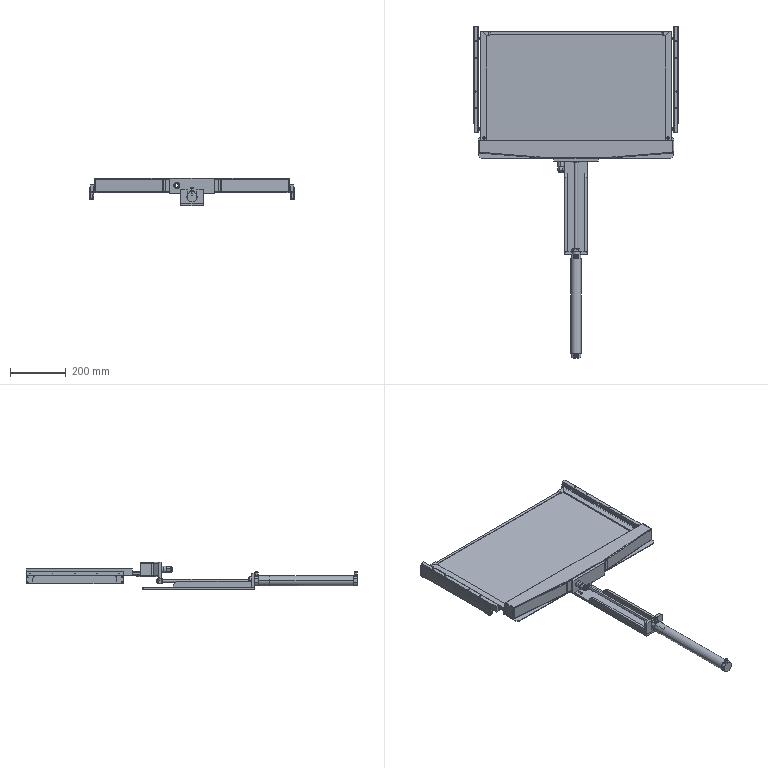Assembly | SolidWorks | mm | 22 component files | 33 solids | 974 faces | box 734 x 1190 x 97 mm | volume 3303453 mm3 | plane 403 | cylinder 333 | cone 192 | torus 22 | spline 16 | sphere 8 | commonest cylinder face diameters 4.5 x44 10 x34 2.5 x28 8 x26 4 x26 3.3 x22 3.4 x20 2.459 x16
Bill of materials:
A4-BPF02-3-PP-L | 4 |  | Short, large-diameter cylinder with chamfered ends. One end face has concentric stepped rings or a recess. A smaller coaxial round shaft sticks out of that face and carries a hex-shaped feature partway along it.
A4-MLCNLSS12-3-L | 1 |  | Hollow round part with a through bore. A hexagonal flats section sits in the middle. A slightly tapered cylindrical spigot with a chamfered end runs from one side. The other side has a short cylindrical neck with a step or groove and a flange-like ring.
A4-MLCNLSS4-1-L | 2 |  | Axially symmetric part with a through bore. From top to bottom: a short cylindrical collar, a narrow groove, a slightly larger ring/flange, a hexagonal body, then a cylindrical shank that tapers slightly and has a chamfer at the lower end.
A4-NA2-N16-L | 1 |  | Long, flat rectangular bar with rounded corners and edges. It has two small through holes near each end.
A4-SDA 32X300-KC-L1 | 1 |  | Long cylindrical rod. Near each end there are flats or notches with small cross holes. One end has a stepped, reduced-diameter tip with a polygonal (hex-like) section.
A4-SDA 32X300-KC-L2 | 1 |  | Long, slender round rod with a short, larger-diameter cylindrical head at one end. The other end has two small collar or hex-like features with a short tip.
AUTO-SpinDryWashing-01-03000001 | 1 | AISI 316 Stainless Steel Sheet (SS) | Elongated flat base plate. One end has an upright block with a U-shaped notch. Two raised rails run along the long edges for part of the length. The thinner opposite end has four slotted holes.
AUTO-SpinDryWashing-01-03000002 | 1 | AISI 316 Stainless Steel Sheet (SS) | Long rectangular box-section beam with rounded edges sitting on a wider flat base flange with chamfered ends. A plate wraps around the middle and carries a projecting cylindrical boss and a tab with a slot below it.
AUTO-SpinDryWashing-01-03000003 | 1 | Glass | Thin, flat rectangular plate with no visible holes or features.
AUTO-SpinDryWashing-01-03000004 | 1 | AISI 316 Stainless Steel Sheet (SS) | Long bar with a stepped, notched cross-section. A row of small holes runs along the top face. Both ends have rebated steps with small holes.
AUTO-SpinDryWashing-01-03000005 | 1 | AISI 304 | Long bar with a channel-like cross-section that has a rectangular groove along one side. Two larger holes sit near one end and small holes near the other. The corners at the ends are chamfered.
AUTO-SpinDryWashing-01-03000006 | 1 | AISI 304 | Long, slender bar with a side-notched cross-section and a round hole visible through the end face. The ends are stepped tabs with small holes and chamfered corners.
AUTO-SpinDryWashing-01-03000007 | 1 | AISI 304 | Long bar with a rectangular groove along one side. Two holes sit near one end. The ends have chamfered corners.
AUTO-SpinDryWashing-01-03000008 | 1 | AISI 304 | Long straight prismatic bar. Its constant cross-section is mostly rectangular, and one long side has a stepped profile: a narrow upper rib, a recessed longitudinal channel, and a lower lip. The top face has a row of small holes.
AUTO-SpinDryWashing-01-03000009 | 2 | AISI 304 | Thin, flat, elongated plate shaped like a shallow U or bridge. A long rectangular cutout along one long edge, with rounded inner corners, leaves a narrow top strip joining two wider end pads. The plate has small holes in the end pads and along the strip.
'- | 1 | AISI 304 | Long straight bar of constant cross-section. The profile is a rectangle with a stepped edge along one side: two projecting lips with a shallow recess between them, running the full length. Holes are spaced along the top face and along one side face.
Mates:
1. coincident | AUTO-SpinDryWashing-01-03000001-1 face at (40, 0, 58) dir (0, -1, 0) | A4-SDA 32X300-KC-L-1/A4-SDA 32X300-KC-L1-1 face at (0, 0, 31) dir (0, 1, 0)
2. concentric | AUTO-SpinDryWashing-01-03000001-1 face at (0, 60, 31) dir (0, -1, 0) r 14.5 | A4-SDA 32X300-KC-L-1/A4-SDA 32X300-KC-L1-1 face at (0, 20, 31) dir (0, -1, 0) r 13.5
3. parallel | AUTO-SpinDryWashing-01-03000001-1 face at (0, 0, 58) dir (0, 0, 1) | A4-SDA 32X300-KC-L-1/A4-SDA 32X300-KC-L1-1 face at (10, 0, 50) dir (0, 0, 1)
4. coincident | AUTO-SpinDryWashing-01-03000002-1 plane at (0, 343, 72) dir (-1, 0, 0) | assembly plane at (0, 0, 0) dir (1, 0, 0)
5. parallel | AUTO-SpinDryWashing-01-03000001-1 face at (40, 0, 58) dir (0, -1, 0) | AUTO-SpinDryWashing-01-03000002-1 face at (0, 333, 72) dir (0, -1, 0)
6. coincident | A4-SDA 32X300-KC-L-1/A4-SDA 32X300-KC-L2-1 face at (0, 343, 31) dir (0, -1, 0) | AUTO-SpinDryWashing-01-03000002-1 face at (0, 343, 72) dir (0, 1, 0)
7. coincident | AUTO-SpinDryWashing-01-03000002-1 face at (0, 343, 47) dir (0, 0, 1) | AUTO-SpinDryWashing-01-03000004-1 face at (-335, 423, 47) dir (0, 0, -1)
8. coincident | AUTO-SpinDryWashing-01-03000002-1 face at (350, 423, 45) dir (0, 1, 0) | AUTO-SpinDryWashing-01-03000004-1 face at (335, 423, 63) dir (0, 1, 0)
9. coincident | AUTO-SpinDryWashing-01-03000004-1 plane at (0, 408, 53) dir (1, 0, 0) | assembly plane at (0, 0, 0) dir (1, 0, 0)
10. coincident | AUTO-SpinDryWashing-01-03000004-1 face at (-335, 388, 60) dir (0, 1, 0) | AUTO-SpinDryWashing-01-03000003-1 face at (-325, 388, 60) dir (0, -1, 0)
11. coincident | AUTO-SpinDryWashing-01-03000004-1 face at (-335, 423, 55) dir (0, 0, 1) | AUTO-SpinDryWashing-01-03000003-1 face at (0, 588, 55) dir (0, 0, -1)
12. coincident | AUTO-SpinDryWashing-01-03000003-1 plane at (0, 588, 55) dir (1, 0, 0) | assembly plane at (0, 0, 0) dir (1, 0, 0)
13. coincident | AUTO-SpinDryWashing-01-03000003-1 face at (325, 788, 60) dir (1, 0, 0) | AUTO-SpinDryWashing-01-03000005-1 face at (325, 798, 63) dir (-1, 0, 0)
14. coincident | AUTO-SpinDryWashing-01-03000003-1 face at (0, 588, 60) dir (0, 0, 1) | AUTO-SpinDryWashing-01-03000005-1 face at (335, 798, 60) dir (0, 0, -1)
15. coincident | AUTO-SpinDryWashing-01-03000003-1 face at (-325, 788, 60) dir (0, 1, 0) | AUTO-SpinDryWashing-01-03000006-1 face at (335, 788, 50) dir (0, -1, 0)
16. coincident | AUTO-SpinDryWashing-01-03000003-1 face at (0, 588, 55) dir (0, 0, -1) | AUTO-SpinDryWashing-01-03000006-1 face at (335, 798, 55) dir (0, 0, 1)
17. coincident | AUTO-SpinDryWashing-01-03000005-1 face at (335, 798, 52) dir (-0.7071, 0.7071, 0) | AUTO-SpinDryWashing-01-03000006-1 face at (335, 798, 50) dir (0.7071, -0.7071, 0)
18. coincident | AUTO-SpinDryWashing-01-03000003-1 face at (-325, 788, 60) dir (-1, 0, 0) | AUTO-SpinDryWashing-01-03000007-1 face at (-325, 378, 63) dir (1, 0, 0)
19. coincident | AUTO-SpinDryWashing-01-03000003-1 face at (0, 588, 55) dir (0, 0, -1) | AUTO-SpinDryWashing-01-03000007-1 face at (-335, 378, 55) dir (0, 0, 1)
20. coincident | AUTO-SpinDryWashing-01-03000006-1 face at (-335, 798, 50) dir (-0.7071, -0.7071, 0) | AUTO-SpinDryWashing-01-03000007-1 face at (-335, 798, 52) dir (0.7071, 0.7071, 0)
21. distance | AUTO-SpinDryWashing-01-03000001-1 face at (-40, 400, 8) dir (0, 1, 0) | AUTO-SpinDryWashing-01-03000008-3 face at (-357, 818, 57.5) dir (0, 1, 0)
22. coincident | AUTO-SpinDryWashing-01-03000009-1 face at (365, 643, 42.5) dir (-1, 0, 0) | A4-NA2-N16-L-1 face at (365, 748, 35) dir (1, 0, 0)
23. coincident | AUTO-SpinDryWashing-01-03000009-1 face at (367, 468, 42.5) dir (0, -1, 0) | A4-NA2-N16-L-1 face at (365, 468, 20) dir (0, -1, 0)
24. coincident | A4-NA2-N16-L-1 face at (365, 818, 20) dir (0, 0, -1) | A4-NA2-N16-L-2 face at (-365, 468, 20) dir (0, 0, -1)
25. coincident | A4-NA2-N16-L-1 face at (365, 818, 50) dir (0, 1, 0) | A4-NA2-N16-L-2 face at (-365, 818, 20) dir (0, 1, 0)
26. distance | AUTO-SpinDryWashing-01-03000008-3 face at (-349, 468, 57.5) dir (1, 0, 0) | AUTO-SpinDryWashing-01-03000007-1 edge at (-335, 798, 65) dir (0, 0, -1)
27. coincident | AUTO-SpinDryWashing-01-03000008-3 face at (-365, 468, 57.5) dir (-1, 0, 0) | AUTO-SpinDryWashing-01-03000009-2 face at (-365, 643, 42.5) dir (1, 0, 0)
28. coincident | AUTO-SpinDryWashing-01-03000008-3 face at (-357, 818, 57.5) dir (0, 1, 0) | AUTO-SpinDryWashing-01-03000009-2 face at (-365, 818, 42.5) dir (0, 1, 0)
29. coincident | AUTO-SpinDryWashing-01-03000008-3 face at (-357, 468, 65) dir (0, 0, 1) | AUTO-SpinDryWashing-01-03000009-2 face at (-365, 643, 65) dir (0, 0, 1)
30. coincident | AUTO-SpinDryWashing-01-03000009-2 face at (-365, 643, 42.5) dir (1, 0, 0) | A4-NA2-N16-L-2 face at (-365, 748, 35) dir (-1, 0, 0)
31. coincident | AUTO-SpinDryWashing-01-03000008-3 face at (-357, 818, 57.5) dir (0, 1, 0) | A4-NA2-N16-L-2 face at (-365, 818, 20) dir (0, 1, 0)
32. coincident | AUTO-SpinDryWashing-01-03000009-2 face at (-365, 643, 20) dir (0, 0, -1) | A4-NA2-N16-L-2 face at (-365, 468, 20) dir (0, 0, -1)
33. distance | AUTO-SpinDryWashing-01-03000002-1 face at (0, 343, 45) dir (0, 0, -1) | AUTO-SpinDryWashing-01-03000001-1 face at (0, 0, 0) dir (0, 0, -1)
34. coincident | AUTO-SpinDryWashing-01-03000002-1 face at (-55, 313, 72) dir (0, -1, 0) | A4-MLCNLSS12-3-L-1 face at (-46.812, 313, 70.489) dir (0, 1, 0)
35. concentric | AUTO-SpinDryWashing-01-03000009-1 face at (367, 813, 44) dir (1, 0, 0) r 2.25 | A4-NA2-N16-L-1 face at (365, 813, 44) dir (-1, 0, 0) r 2.3
36. concentric | AUTO-SpinDryWashing-01-03000009-1 face at (367, 813, 26) dir (1, 0, 0) r 2.25 | A4-NA2-N16-L-1 face at (352, 813, 26) dir (-1, 0, 0) r 2.15
37. coincident | AUTO-SpinDryWashing-01-03000007-1 face at (-343, 378, 62.75) dir (0, 0, -1) | AUTO-SpinDryWashing-01-03000008-3 face at (-357, 468, 62.75) dir (0, 0, -1)
38. distance | AUTO-SpinDryWashing-01-03000009-1 face at (367, 643, 42.5) dir (1, 0, 0) | AUTO-SpinDryWashing-01-03000009-2 face at (-367, 643, 42.5) dir (-1, 0, 0)
39. coincident | AUTO-SpinDryWashing-01-03000009-1 face at (365, 643, 42.5) dir (-1, 0, 0) | AUTO-SpinDryWashing-01-03000010-5 face at (365, 468, 57.5) dir (1, 0, 0)
40. coincident | AUTO-SpinDryWashing-01-03000008-3 face at (-357, 643, 74) dir (0, 0, 1) | AUTO-SpinDryWashing-01-03000010-5 face at (357, 643, 74) dir (0, 0, 1)
41. coincident | AUTO-SpinDryWashing-01-03000008-3 face at (-357, 818, 57.5) dir (0, 1, 0) | AUTO-SpinDryWashing-01-03000010-5 face at (357, 818, 57.5) dir (0, 1, 0)
42. coincident | AUTO-SpinDryWashing-01-03000005-1 face at (343, 798, 65) dir (0, 1, 0) | AUTO-SpinDryWashing-01-03000006-1 face at (335, 798, 50) dir (0, 1, 0)
43. coincident | A4-SDA 32X300-KC-L-1/A4-SDA 32X300-KC-L1-1 face at (10, 0, 50) dir (0, 0, 1) | A4-MLCNLSS4-1-L-1 face at (-0.2817, -3.615, 50) dir (0, 0, -1)
44. concentric | A4-SDA 32X300-KC-L-1/A4-SDA 32X300-KC-L1-1 face at (0, -8, 50) dir (0, 0, 1) r 4.4 | A4-MLCNLSS4-1-L-1 face at (0, -8, 50) dir (0, 0, -1) r 31.241
45. coincident | A4-SDA 32X300-KC-L-1/A4-SDA 32X300-KC-L1-1 face at (-10, -372, 50) dir (0, 0, 1) | A4-MLCNLSS4-1-L-2 face at (-0.2817, -359.615, 50) dir (0, 0, -1)
46. concentric | A4-SDA 32X300-KC-L-1/A4-SDA 32X300-KC-L1-1 face at (0, -364, 50) dir (0, 0, 1) r 4.4 | A4-MLCNLSS4-1-L-2 face at (0, -364, 50) dir (0, 0, -1) r 31.241
47. concentric | AUTO-SpinDryWashing-01-03000002-1 face at (-55, 313, 72) dir (0, 1, 0) r 31.206 | A4-MLCNLSS12-3-L-1 face at (-55, 313, 72) dir (0, 1, 0) r 31.241
48. coincident | AUTO-SpinDryWashing-01-03000007-1 face at (-339, 378, 52.25) dir (-1, 0, 0) | A4-BPF02-3-PP-L-1 face at (-339, 773, 57.5) dir (1, 0, 0)
49. concentric | AUTO-SpinDryWashing-01-03000007-1 face at (-339, 773, 57.5) dir (-1, 0, 0) r 1.25 | A4-BPF02-3-PP-L-1 face at (-346, 773, 57.5) dir (-1, 0, 0) r 1.23
50. concentric | AUTO-SpinDryWashing-01-03000008-3 face at (-353, 448, 57.75) dir (1, 0, 0) r 1.25 | A4-BPF02-3-PP-L-2 face at (-346, 448, 57.75) dir (1, 0, 0) r 1.23
51. coincident | AUTO-SpinDryWashing-01-03000008-3 face at (-353, 468, 57.5) dir (1, 0, 0) | A4-BPF02-3-PP-L-2 face at (-353, 448, 57.75) dir (-1, 0, 0)
52. coincident | AUTO-SpinDryWashing-01-03000005-1 face at (339, 378, 62.75) dir (1, 0, 0) | A4-BPF02-3-PP-L-3 face at (339, 773, 57.5) dir (-1, 0, 0)
53. concentric | AUTO-SpinDryWashing-01-03000005-1 face at (339, 773, 57.5) dir (1, 0, 0) r 1.25 | A4-BPF02-3-PP-L-3 face at (346, 773, 57.5) dir (1, 0, 0) r 1.23
54. coincident | AUTO-SpinDryWashing-01-03000010-5 face at (353, 468, 57.5) dir (-1, 0, 0) | A4-BPF02-3-PP-L-4 face at (353, 448, 57.75) dir (1, 0, 0)
55. concentric | AUTO-SpinDryWashing-01-03000010-5 face at (353, 448, 57.75) dir (-1, 0, 0) r 1.25 | A4-BPF02-3-PP-L-4 face at (346, 448, 57.75) dir (-1, 0, 0) r 1.23
56. concentric | A4-SDA 32X300-KC-L1-1 face at (0, 0, -340) dir (0, 0, 1) r 18 | A4-SDA 32X300-KC-L2-1 face at (0, 0, -340) dir (0, 0, 1) r 16
57. distance | A4-SDA 32X300-KC-L2-1 face at (0, 0, -340) dir (0, 0, -1) | A4-SDA 32X300-KC-L1-1 face at (0, 0, -340) dir (0, 0, 1)